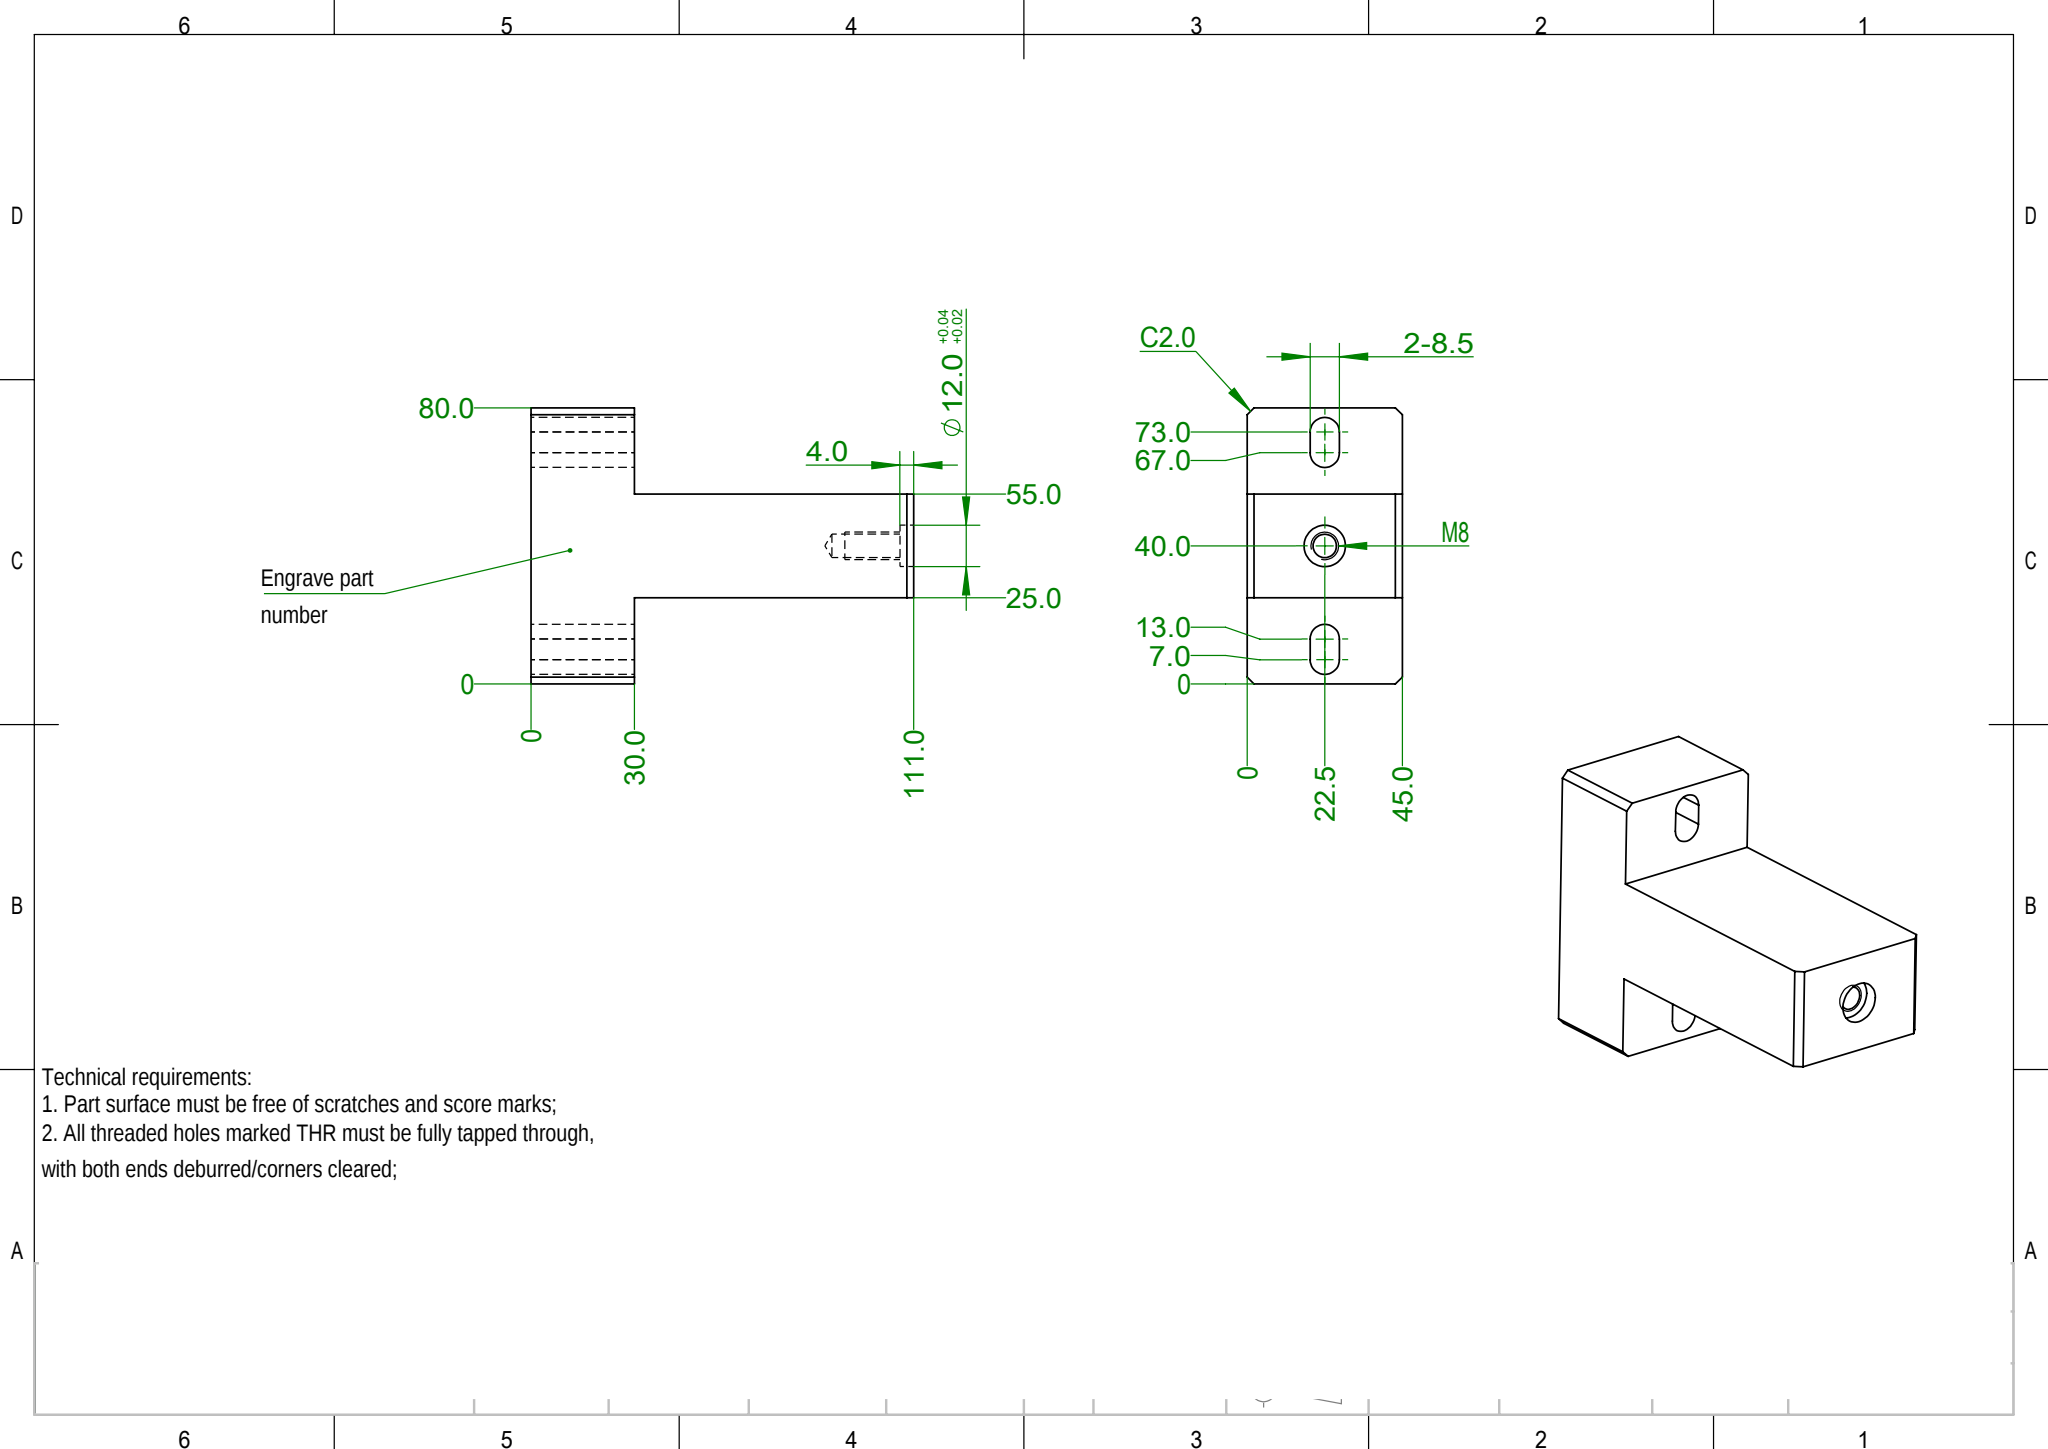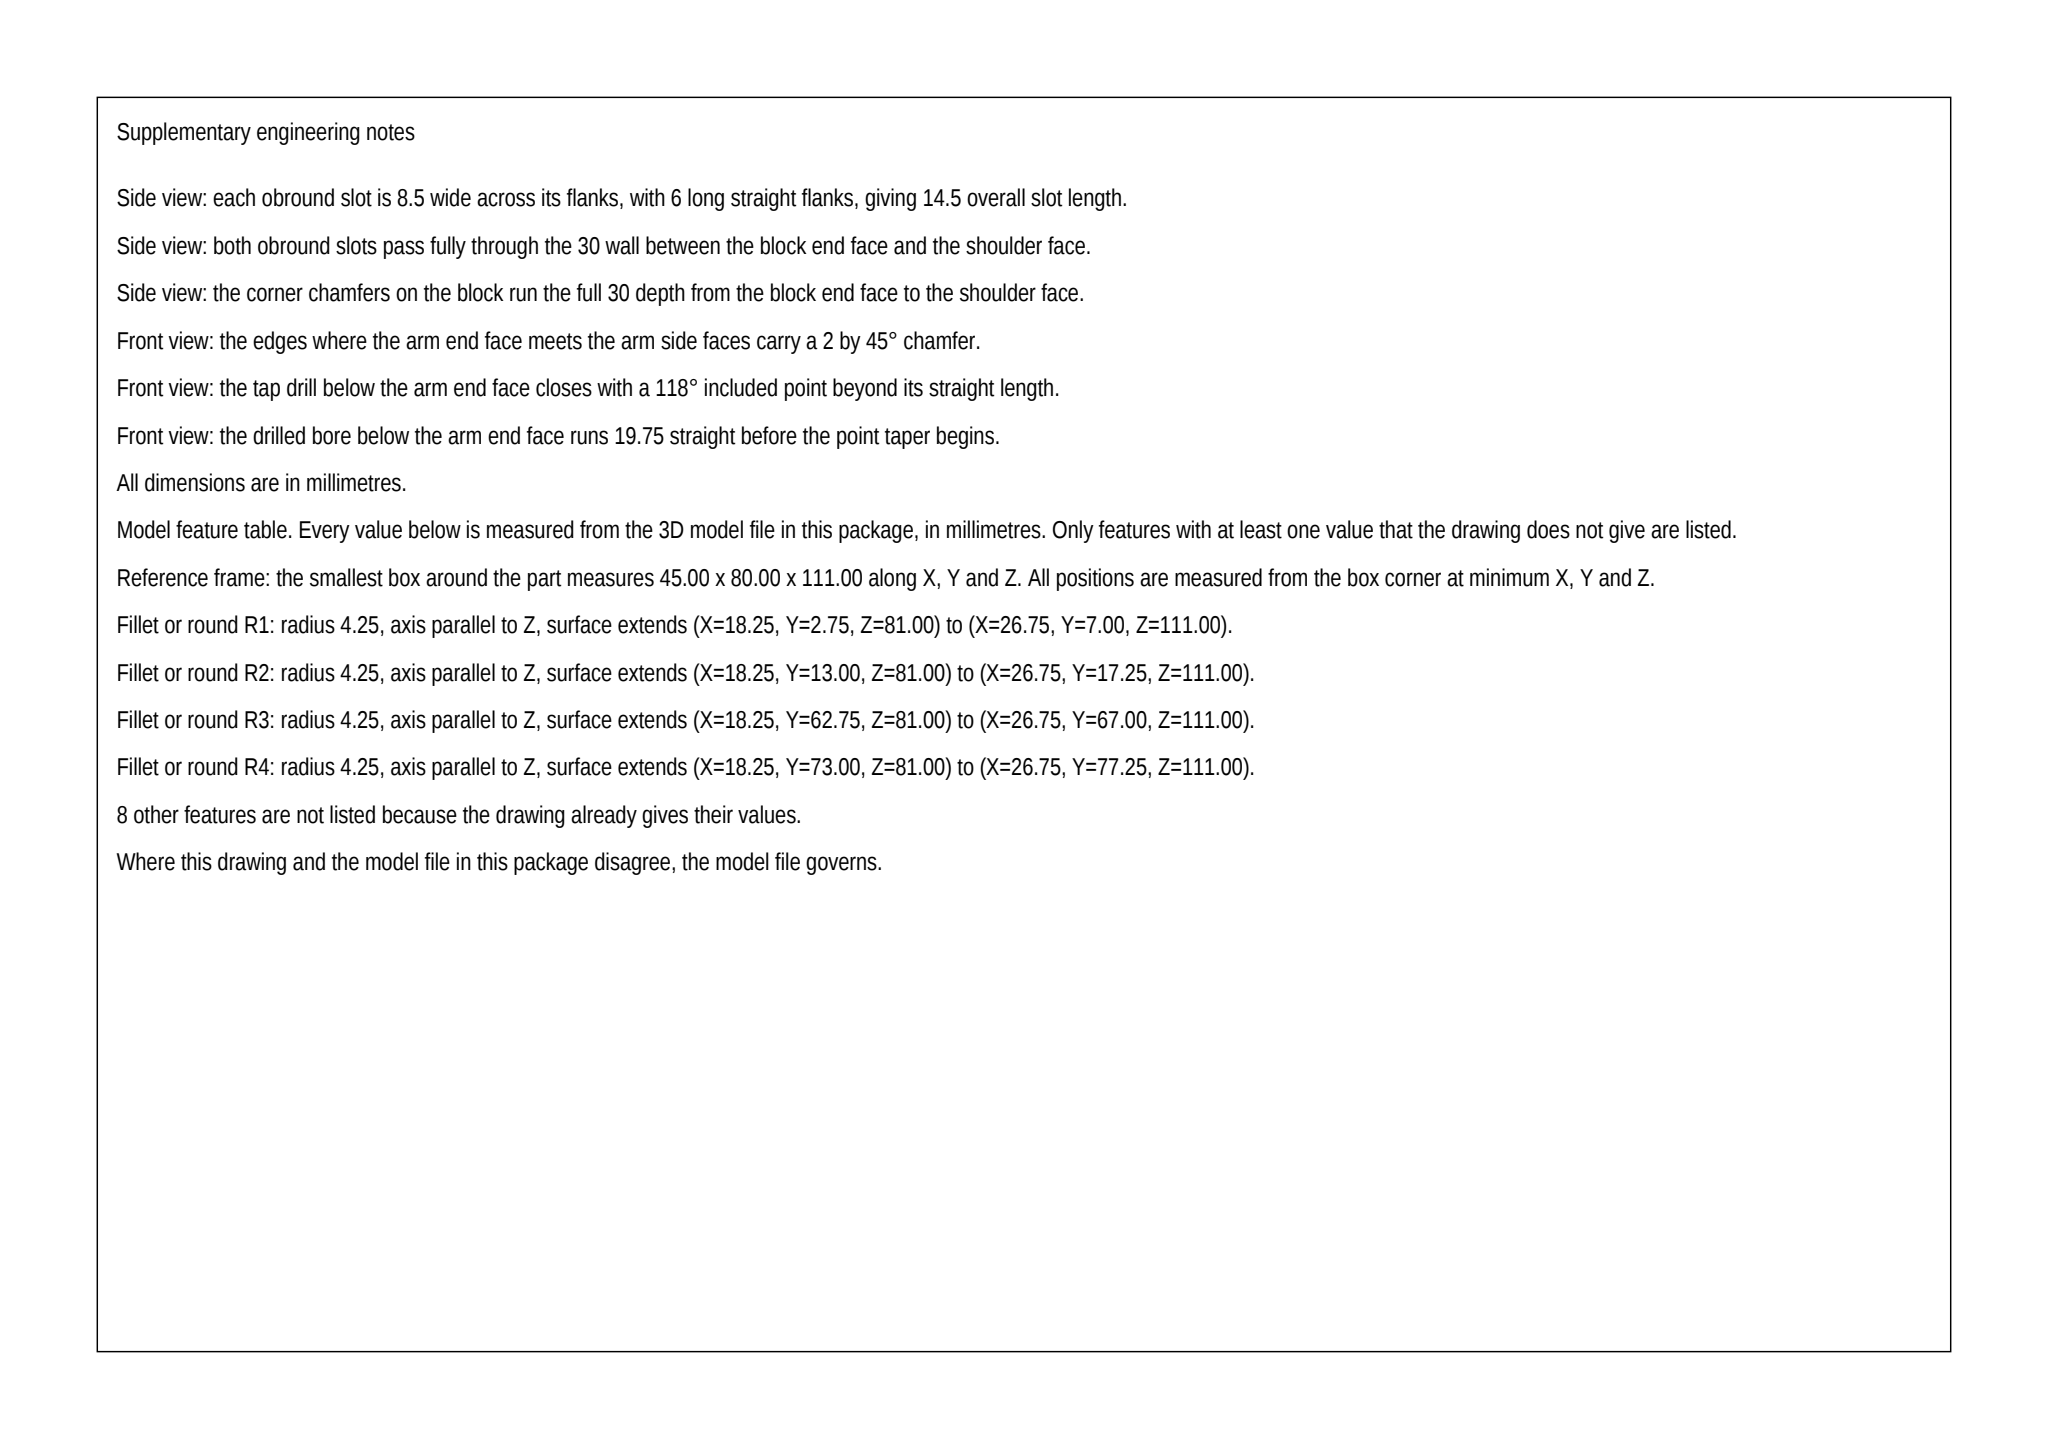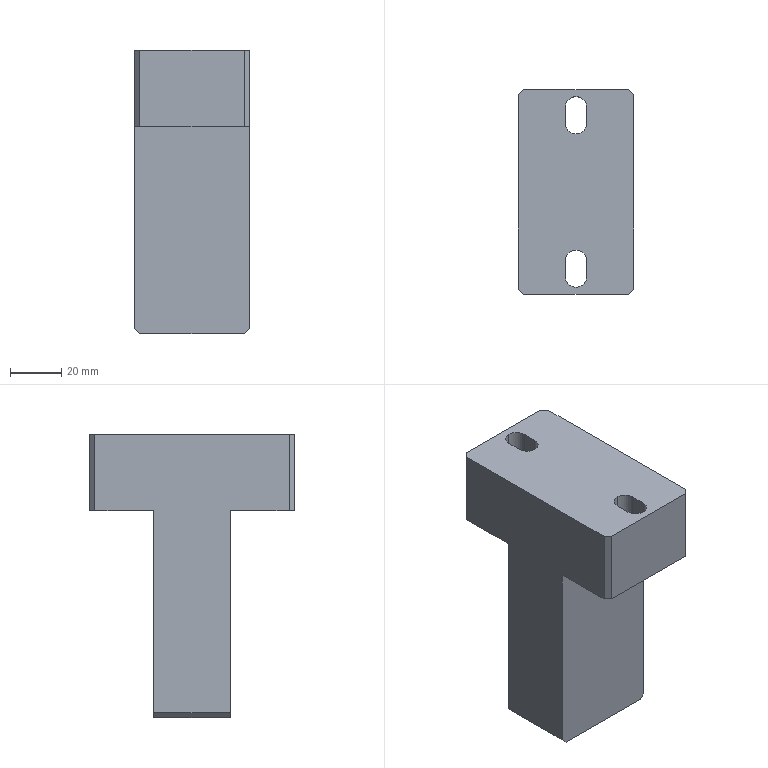Part | SolidWorks | mm | 1 solid | 33 faces | box 45 x 80 x 111 mm | volume 209331 mm3 | plane 21 | cylinder 10 | cone 2 | commonest cylinder face diameters 8.5 x6 6.8 x2 12 x2
build123d program:
from build123d import *

# Parameters (mm, degrees)
SKETCH1_W             = 45
SKETCH1_H             = 80
BOSS_EXTRUDE1_DEPTH   = 111
SKETCH2_R             = 6
CUT_EXTRUDE1_DEPTH    = 4
M8_TAPPED_HOLE1_D     = 6.8
M8_TAPPED_HOLE1_DEPTH = 19.75
M8_TAPPED_HOLE1_TIP   = 2.043
SKETCH5_W             = 126.295
SKETCH5_H             = 86.94
CUT_EXTRUDE2_DEPTH    = 111
CUT_EXTRUDE3_DEPTH    = 111
CHAMFER1_SIZE         = 2
CHAMFER2_SIZE         = 2


with BuildPart() as part:
    # Sketch1 → Boss-Extrude1 (new body)
    with BuildSketch(Plane.XY):
        Rectangle(SKETCH1_W, SKETCH1_H)
    extrude(amount=BOSS_EXTRUDE1_DEPTH)

    # Sketch2 → Cut-Extrude1 (cut)
    with BuildSketch(Plane(origin=(0, 0, 0), x_dir=(-1, 0, 0), z_dir=(0, 0, -1))):
        Circle(SKETCH2_R)
    extrude(amount=-CUT_EXTRUDE1_DEPTH, mode=Mode.SUBTRACT)

    # M8 Tapped Hole1
    with Locations(Plane(origin=(0, 0, 4), x_dir=(-1, 0, 0), z_dir=(0, 0, -1))):
        with Locations((0, 0)):
            Hole(M8_TAPPED_HOLE1_D / 2, depth=M8_TAPPED_HOLE1_DEPTH)
            with Locations((0, 0, -(M8_TAPPED_HOLE1_DEPTH + M8_TAPPED_HOLE1_TIP / 2))):  # 118° drill point
                Cone(0, M8_TAPPED_HOLE1_D / 2, M8_TAPPED_HOLE1_TIP, mode=Mode.SUBTRACT)

    # Sketch5 → Cut-Extrude2 (cut)
    with BuildSketch(Plane(origin=(22.5, 0, 0), x_dir=(0, 0, -1), z_dir=(1, 0, 0))):
        with Locations((-17.853, 58.47)):
            Rectangle(SKETCH5_W, SKETCH5_H)
    cut_extrude2 = extrude(amount=-CUT_EXTRUDE2_DEPTH, mode=Mode.SUBTRACT)

    # Sketch7 → Cut-Extrude3 (cut)
    with BuildSketch(Plane(origin=(0, 0, 81), x_dir=(-1, 0, 0), z_dir=(0, 0, -1))):
        with BuildLine():
            Line((-4.25, 27), (-4.25, 33))
            ThreePointArc((-4.25, 33), (0, 37.25), (4.25, 33))
            Line((4.25, 33), (4.25, 27))
            ThreePointArc((4.25, 27), (0, 22.75), (-4.25, 27))
        make_face()
    cut_extrude3 = extrude(amount=-CUT_EXTRUDE3_DEPTH, mode=Mode.SUBTRACT)

    # Mirror1: Cut-Extrude2, Cut-Extrude3 across plane
    add(cut_extrude2.mirror(Plane.ZX), mode=Mode.SUBTRACT)
    add(cut_extrude3.mirror(Plane.ZX), mode=Mode.SUBTRACT)

    # Chamfer1
    chamfer1_edges = [part.edges().sort_by_distance(p)[0] for p in [
        (-22.5, 40, 96),
        (22.5, 40, 96),
        (22.5, -40, 96),
        (-22.5, -40, 96),
    ]]
    chamfer(chamfer1_edges, length=CHAMFER1_SIZE)

    # Chamfer2
    chamfer2_edges = [part.edges().sort_by_distance(p)[0] for p in [
        (-22.5, 0, 0),
        (22.5, 0, 0),
    ]]
    chamfer(chamfer2_edges, length=CHAMFER2_SIZE)


solid = part.part